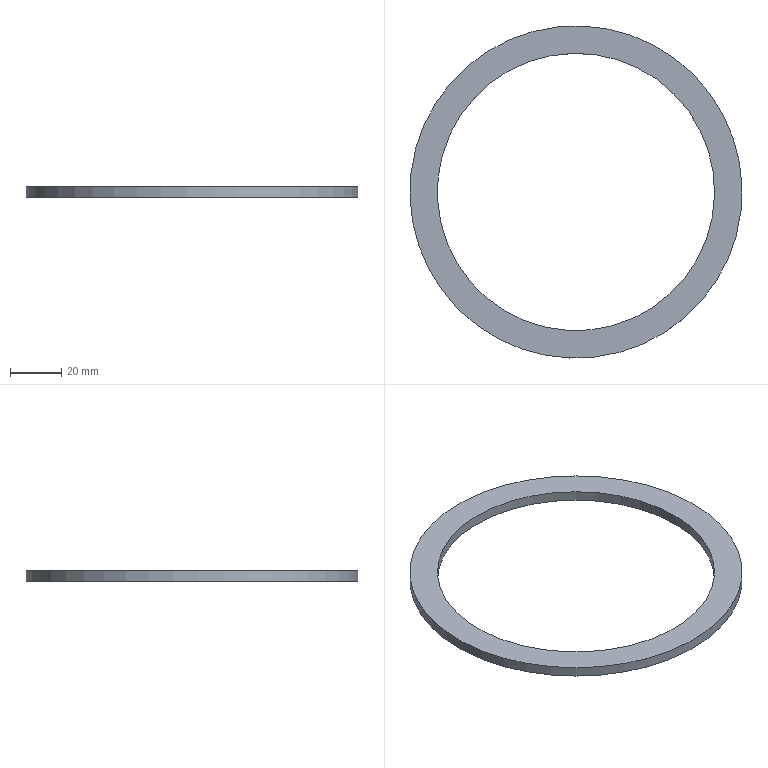Component | NX | CA6140-ZHUZHOU-DANGYOU | 1 solid | 4 faces | box 130 x 130 x 4 mm | volume 16109 mm3 | cylinder 2 | plane 2 | commonest cylinder face diameters 130 x1 108.5 x1
STEP:
#1=CARTESIAN_POINT('',(0.,0.,0.));
#2=DIRECTION('',(0.,0.,1.));
#3=DIRECTION('',(1.,0.,0.));
#4=AXIS2_PLACEMENT_3D('',#1,#2,#3);
#5=CARTESIAN_POINT('',(45.962,45.962,67.049));
#6=VERTEX_POINT('',#5);
#7=CARTESIAN_POINT('',(0.,-0.,67.049));
#8=DIRECTION('',(0.,0.,-1.));
#9=DIRECTION('',(0.7071,0.7071,0.));
#10=AXIS2_PLACEMENT_3D('',#7,#8,#9);
#11=CIRCLE('',#10,65.);
#12=CARTESIAN_POINT('',(0.,-0.,67.049));
#13=DIRECTION('',(0.,0.,-1.));
#14=DIRECTION('',(-0.7071,-0.7071,0.));
#15=AXIS2_PLACEMENT_3D('',#12,#13,#14);
#16=CYLINDRICAL_SURFACE('',#15,65.);
#17=CARTESIAN_POINT('',(3.142,0.));
#18=DIRECTION('',(1.,0.));
#19=VECTOR('',#18,1.);
#20=LINE('',#17,#19);
#21=(GEOMETRIC_REPRESENTATION_CONTEXT(2)PARAMETRIC_REPRESENTATION_CONTEXT()REPRESENTATION_CONTEXT('',''));
#22=DEFINITIONAL_REPRESENTATION('',(#20),#21);
#23=PCURVE('',#16,#22);
#24=CARTESIAN_POINT('',(0.,-0.,67.049));
#25=DIRECTION('',(0.,0.,-1.));
#26=DIRECTION('',(-0.7071,-0.7071,0.));
#27=AXIS2_PLACEMENT_3D('',#24,#25,#26);
#28=PLANE('',#27);
#29=CARTESIAN_POINT('',(0.,0.));
#30=DIRECTION('',(-1.,0.));
#31=AXIS2_PLACEMENT_2D('',#29,#30);
#32=CIRCLE('',#31,65.);
#33=(GEOMETRIC_REPRESENTATION_CONTEXT(2)PARAMETRIC_REPRESENTATION_CONTEXT()REPRESENTATION_CONTEXT('',''));
#34=DEFINITIONAL_REPRESENTATION('',(#32),#33);
#35=PCURVE('',#28,#34);
#36=SURFACE_CURVE('',#11,(#23,#35),.PCURVE_S1.);
#37=EDGE_CURVE('',#6,#6,#36,.T.);
#38=ORIENTED_EDGE('',*,*,#37,.T.);
#39=CARTESIAN_POINT('',(45.962,45.962,63.049));
#40=VERTEX_POINT('',#39);
#41=CARTESIAN_POINT('',(45.962,45.962,67.049));
#42=CARTESIAN_POINT('',(45.962,45.962,63.049));
#43=B_SPLINE_CURVE_WITH_KNOTS('',1,(#41,#42),.UNSPECIFIED.,.F.,.F.,(2,2),(0.,4.),.PIECEWISE_BEZIER_KNOTS.);
#44=CARTESIAN_POINT('',(9.425,0.));
#45=DIRECTION('',(0.,1.));
#46=VECTOR('',#45,1.);
#47=LINE('',#44,#46);
#48=(GEOMETRIC_REPRESENTATION_CONTEXT(2)PARAMETRIC_REPRESENTATION_CONTEXT()REPRESENTATION_CONTEXT('',''));
#49=DEFINITIONAL_REPRESENTATION('',(#47),#48);
#50=PCURVE('',#16,#49);
#51=CARTESIAN_POINT('',(3.142,0.));
#52=DIRECTION('',(0.,1.));
#53=VECTOR('',#52,1.);
#54=LINE('',#51,#53);
#55=(GEOMETRIC_REPRESENTATION_CONTEXT(2)PARAMETRIC_REPRESENTATION_CONTEXT()REPRESENTATION_CONTEXT('',''));
#56=DEFINITIONAL_REPRESENTATION('',(#54),#55);
#57=PCURVE('',#16,#56);
#58=SEAM_CURVE('',#43,(#50,#57),.PCURVE_S1.);
#59=EDGE_CURVE('',#6,#40,#58,.T.);
#60=ORIENTED_EDGE('',*,*,#59,.T.);
#61=CARTESIAN_POINT('',(0.,-0.,63.049));
#62=DIRECTION('',(0.,0.,-1.));
#63=DIRECTION('',(0.7071,0.7071,0.));
#64=AXIS2_PLACEMENT_3D('',#61,#62,#63);
#65=CIRCLE('',#64,65.);
#66=CARTESIAN_POINT('',(3.142,4.));
#67=DIRECTION('',(1.,0.));
#68=VECTOR('',#67,1.);
#69=LINE('',#66,#68);
#70=(GEOMETRIC_REPRESENTATION_CONTEXT(2)PARAMETRIC_REPRESENTATION_CONTEXT()REPRESENTATION_CONTEXT('',''));
#71=DEFINITIONAL_REPRESENTATION('',(#69),#70);
#72=PCURVE('',#16,#71);
#73=CARTESIAN_POINT('',(0.,-0.,63.049));
#74=DIRECTION('',(0.,0.,-1.));
#75=DIRECTION('',(-0.7071,-0.7071,0.));
#76=AXIS2_PLACEMENT_3D('',#73,#74,#75);
#77=PLANE('',#76);
#78=CARTESIAN_POINT('',(0.,0.));
#79=DIRECTION('',(-1.,0.));
#80=AXIS2_PLACEMENT_2D('',#78,#79);
#81=CIRCLE('',#80,65.);
#82=(GEOMETRIC_REPRESENTATION_CONTEXT(2)PARAMETRIC_REPRESENTATION_CONTEXT()REPRESENTATION_CONTEXT('',''));
#83=DEFINITIONAL_REPRESENTATION('',(#81),#82);
#84=PCURVE('',#77,#83);
#85=SURFACE_CURVE('',#65,(#72,#84),.PCURVE_S1.);
#86=EDGE_CURVE('',#40,#40,#85,.T.);
#87=ORIENTED_EDGE('',*,*,#86,.F.);
#88=ORIENTED_EDGE('',*,*,#59,.F.);
#89=EDGE_LOOP('',(#38,#60,#87,#88));
#90=FACE_BOUND('',#89,.T.);
#91=ADVANCED_FACE('',(#90),#16,.T.);
#92=CARTESIAN_POINT('',(38.361,38.361,67.049));
#93=VERTEX_POINT('',#92);
#94=CARTESIAN_POINT('',(0.,-0.,67.049));
#95=DIRECTION('',(0.,0.,-1.));
#96=DIRECTION('',(0.7071,0.7071,0.));
#97=AXIS2_PLACEMENT_3D('',#94,#95,#96);
#98=CIRCLE('',#97,54.25);
#99=CARTESIAN_POINT('',(0.,-0.,67.049));
#100=DIRECTION('',(0.,0.,-1.));
#101=DIRECTION('',(-0.7071,-0.7071,0.));
#102=AXIS2_PLACEMENT_3D('',#99,#100,#101);
#103=CYLINDRICAL_SURFACE('',#102,54.25);
#104=CARTESIAN_POINT('',(3.142,0.));
#105=DIRECTION('',(1.,0.));
#106=VECTOR('',#105,1.);
#107=LINE('',#104,#106);
#108=(GEOMETRIC_REPRESENTATION_CONTEXT(2)PARAMETRIC_REPRESENTATION_CONTEXT()REPRESENTATION_CONTEXT('',''));
#109=DEFINITIONAL_REPRESENTATION('',(#107),#108);
#110=PCURVE('',#103,#109);
#111=CARTESIAN_POINT('',(0.,0.));
#112=DIRECTION('',(-1.,0.));
#113=AXIS2_PLACEMENT_2D('',#111,#112);
#114=CIRCLE('',#113,54.25);
#115=(GEOMETRIC_REPRESENTATION_CONTEXT(2)PARAMETRIC_REPRESENTATION_CONTEXT()REPRESENTATION_CONTEXT('',''));
#116=DEFINITIONAL_REPRESENTATION('',(#114),#115);
#117=PCURVE('',#28,#116);
#118=SURFACE_CURVE('',#98,(#110,#117),.PCURVE_S1.);
#119=EDGE_CURVE('',#93,#93,#118,.T.);
#120=ORIENTED_EDGE('',*,*,#119,.T.);
#121=CARTESIAN_POINT('',(38.361,38.361,63.049));
#122=VERTEX_POINT('',#121);
#123=CARTESIAN_POINT('',(38.361,38.361,67.049));
#124=CARTESIAN_POINT('',(38.361,38.361,63.049));
#125=B_SPLINE_CURVE_WITH_KNOTS('',1,(#123,#124),.UNSPECIFIED.,.F.,.F.,(2,2),(0.,4.),.PIECEWISE_BEZIER_KNOTS.);
#126=CARTESIAN_POINT('',(9.425,0.));
#127=DIRECTION('',(0.,1.));
#128=VECTOR('',#127,1.);
#129=LINE('',#126,#128);
#130=(GEOMETRIC_REPRESENTATION_CONTEXT(2)PARAMETRIC_REPRESENTATION_CONTEXT()REPRESENTATION_CONTEXT('',''));
#131=DEFINITIONAL_REPRESENTATION('',(#129),#130);
#132=PCURVE('',#103,#131);
#133=CARTESIAN_POINT('',(3.142,0.));
#134=DIRECTION('',(0.,1.));
#135=VECTOR('',#134,1.);
#136=LINE('',#133,#135);
#137=(GEOMETRIC_REPRESENTATION_CONTEXT(2)PARAMETRIC_REPRESENTATION_CONTEXT()REPRESENTATION_CONTEXT('',''));
#138=DEFINITIONAL_REPRESENTATION('',(#136),#137);
#139=PCURVE('',#103,#138);
#140=SEAM_CURVE('',#125,(#132,#139),.PCURVE_S1.);
#141=EDGE_CURVE('',#93,#122,#140,.T.);
#142=ORIENTED_EDGE('',*,*,#141,.T.);
#143=CARTESIAN_POINT('',(0.,-0.,63.049));
#144=DIRECTION('',(0.,0.,-1.));
#145=DIRECTION('',(0.7071,0.7071,0.));
#146=AXIS2_PLACEMENT_3D('',#143,#144,#145);
#147=CIRCLE('',#146,54.25);
#148=CARTESIAN_POINT('',(3.142,4.));
#149=DIRECTION('',(1.,0.));
#150=VECTOR('',#149,1.);
#151=LINE('',#148,#150);
#152=(GEOMETRIC_REPRESENTATION_CONTEXT(2)PARAMETRIC_REPRESENTATION_CONTEXT()REPRESENTATION_CONTEXT('',''));
#153=DEFINITIONAL_REPRESENTATION('',(#151),#152);
#154=PCURVE('',#103,#153);
#155=CARTESIAN_POINT('',(0.,0.));
#156=DIRECTION('',(-1.,0.));
#157=AXIS2_PLACEMENT_2D('',#155,#156);
#158=CIRCLE('',#157,54.25);
#159=(GEOMETRIC_REPRESENTATION_CONTEXT(2)PARAMETRIC_REPRESENTATION_CONTEXT()REPRESENTATION_CONTEXT('',''));
#160=DEFINITIONAL_REPRESENTATION('',(#158),#159);
#161=PCURVE('',#77,#160);
#162=SURFACE_CURVE('',#147,(#154,#161),.PCURVE_S1.);
#163=EDGE_CURVE('',#122,#122,#162,.T.);
#164=ORIENTED_EDGE('',*,*,#163,.F.);
#165=ORIENTED_EDGE('',*,*,#141,.F.);
#166=EDGE_LOOP('',(#120,#142,#164,#165));
#167=FACE_BOUND('',#166,.F.);
#168=ADVANCED_FACE('',(#167),#103,.F.);
#169=ORIENTED_EDGE('',*,*,#37,.F.);
#170=EDGE_LOOP('',(#169));
#171=FACE_BOUND('',#170,.T.);
#172=ORIENTED_EDGE('',*,*,#119,.T.);
#173=EDGE_LOOP('',(#172));
#174=FACE_BOUND('',#173,.T.);
#175=ADVANCED_FACE('',(#171,#174),#28,.F.);
#176=ORIENTED_EDGE('',*,*,#86,.T.);
#177=EDGE_LOOP('',(#176));
#178=FACE_BOUND('',#177,.T.);
#179=ORIENTED_EDGE('',*,*,#163,.F.);
#180=EDGE_LOOP('',(#179));
#181=FACE_BOUND('',#180,.T.);
#182=ADVANCED_FACE('',(#178,#181),#77,.T.);
#183=CLOSED_SHELL('',(#91,#168,#175,#182));
#184=MANIFOLD_SOLID_BREP('',#183);
#185=(LENGTH_UNIT()NAMED_UNIT(*)SI_UNIT(.MILLI.,.METRE.));
#186=UNCERTAINTY_MEASURE_WITH_UNIT(LENGTH_MEASURE(0.00001),#185,'','');
#187=(NAMED_UNIT(*)PLANE_ANGLE_UNIT()SI_UNIT($,.RADIAN.));
#188=(NAMED_UNIT(*)SI_UNIT($,.STERADIAN.)SOLID_ANGLE_UNIT());
#189=(GEOMETRIC_REPRESENTATION_CONTEXT(3)GLOBAL_UNCERTAINTY_ASSIGNED_CONTEXT((#186))GLOBAL_UNIT_ASSIGNED_CONTEXT((#185,#187,#188))REPRESENTATION_CONTEXT('',''));
#190=ADVANCED_BREP_SHAPE_REPRESENTATION('',(#4,#184),#189);